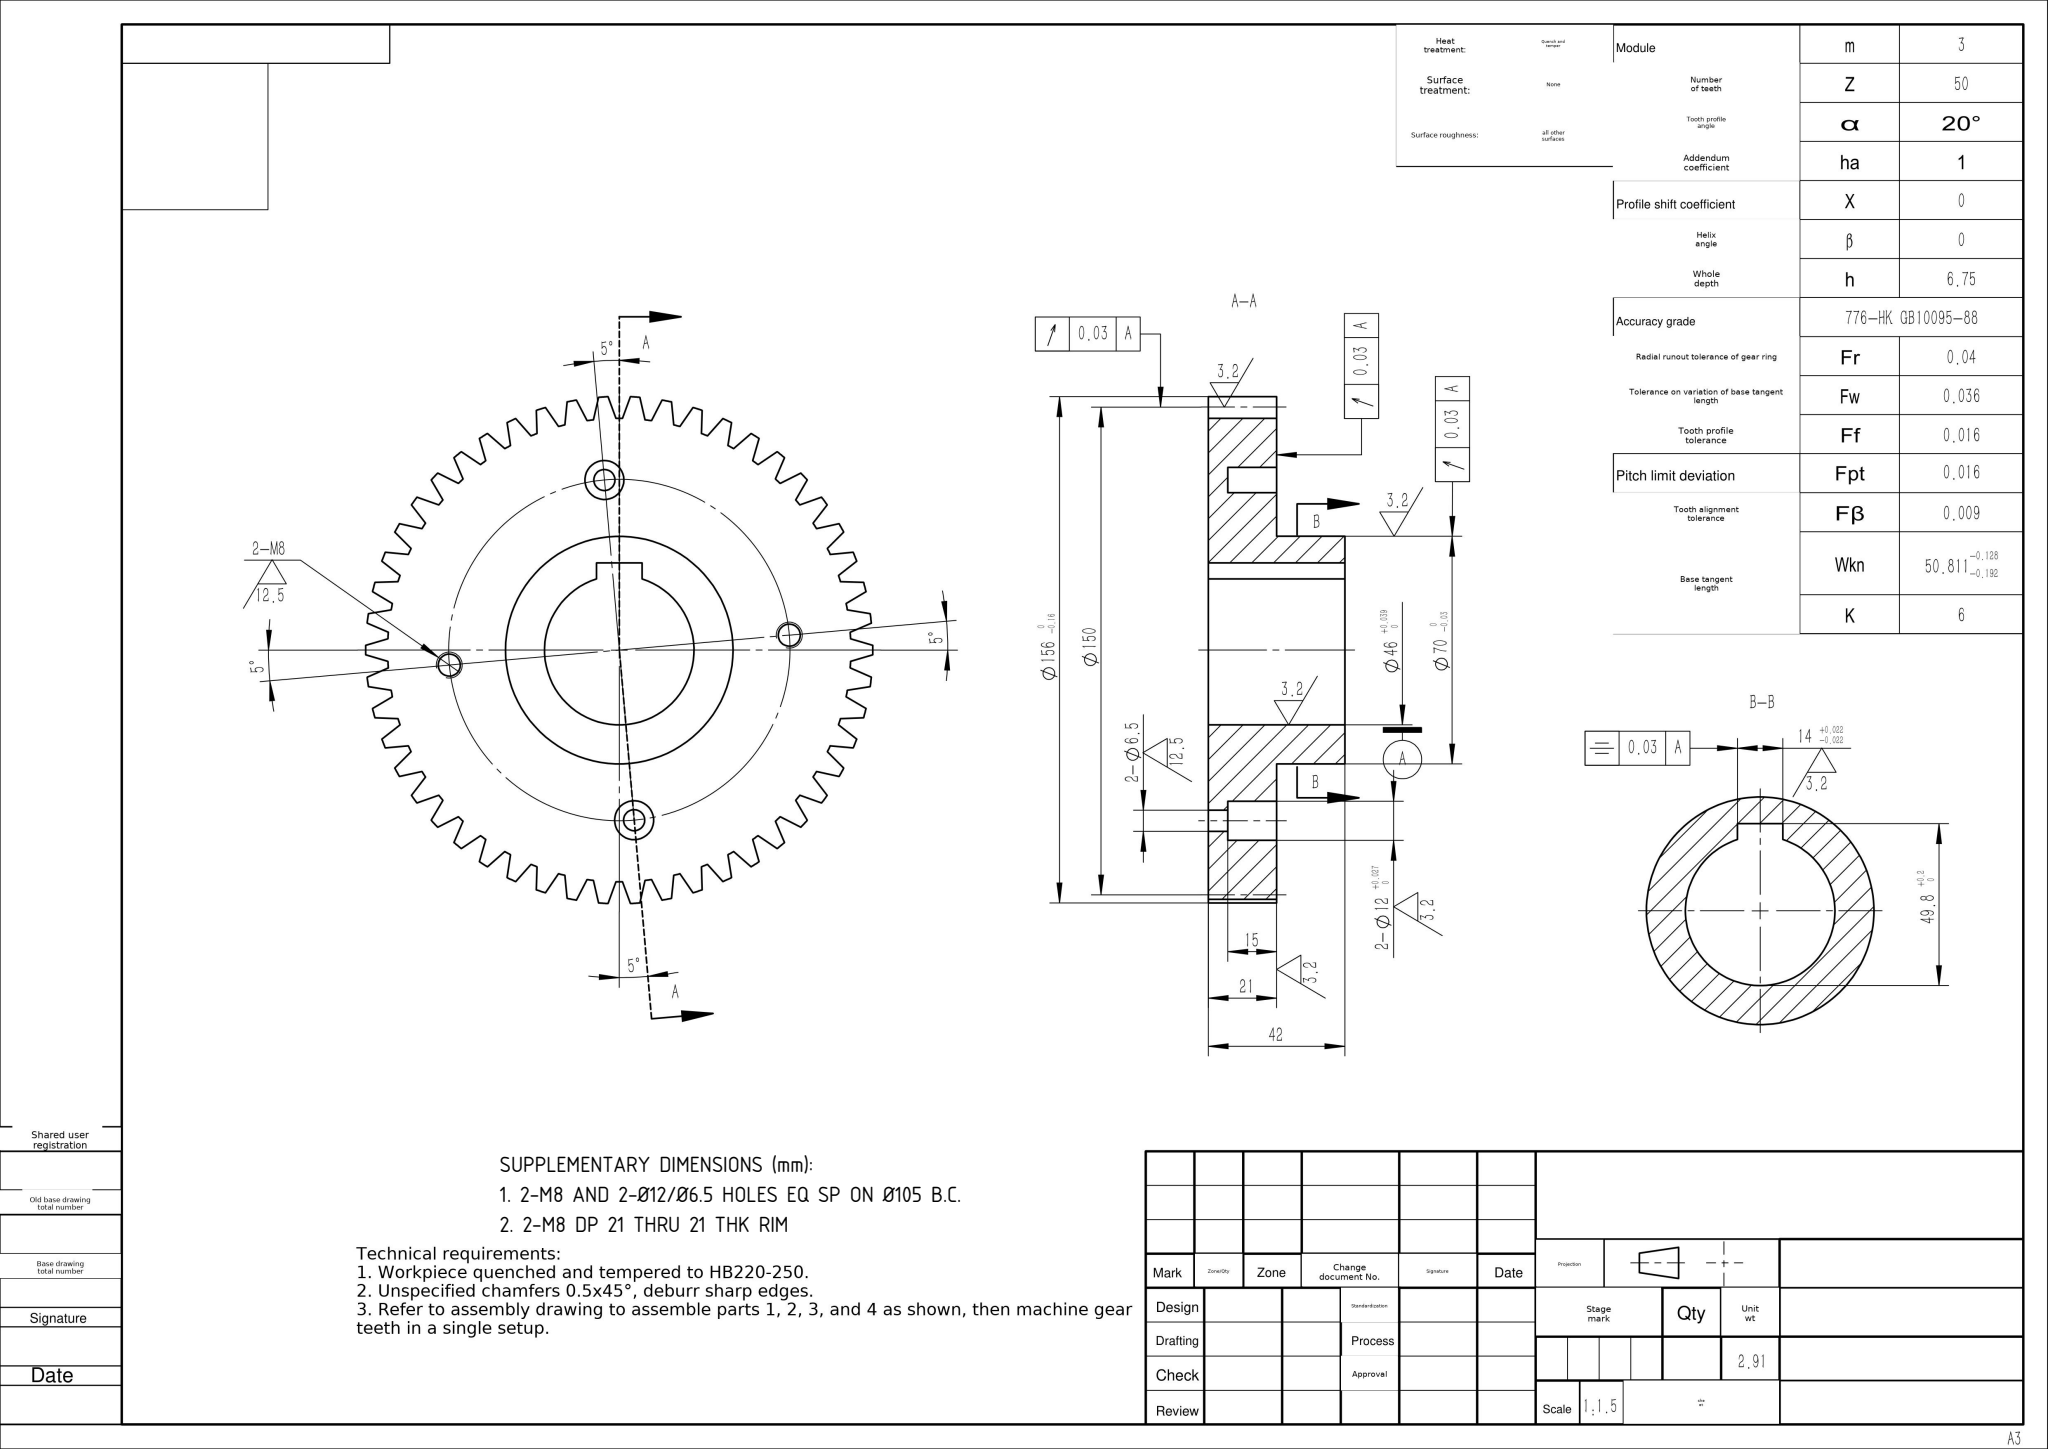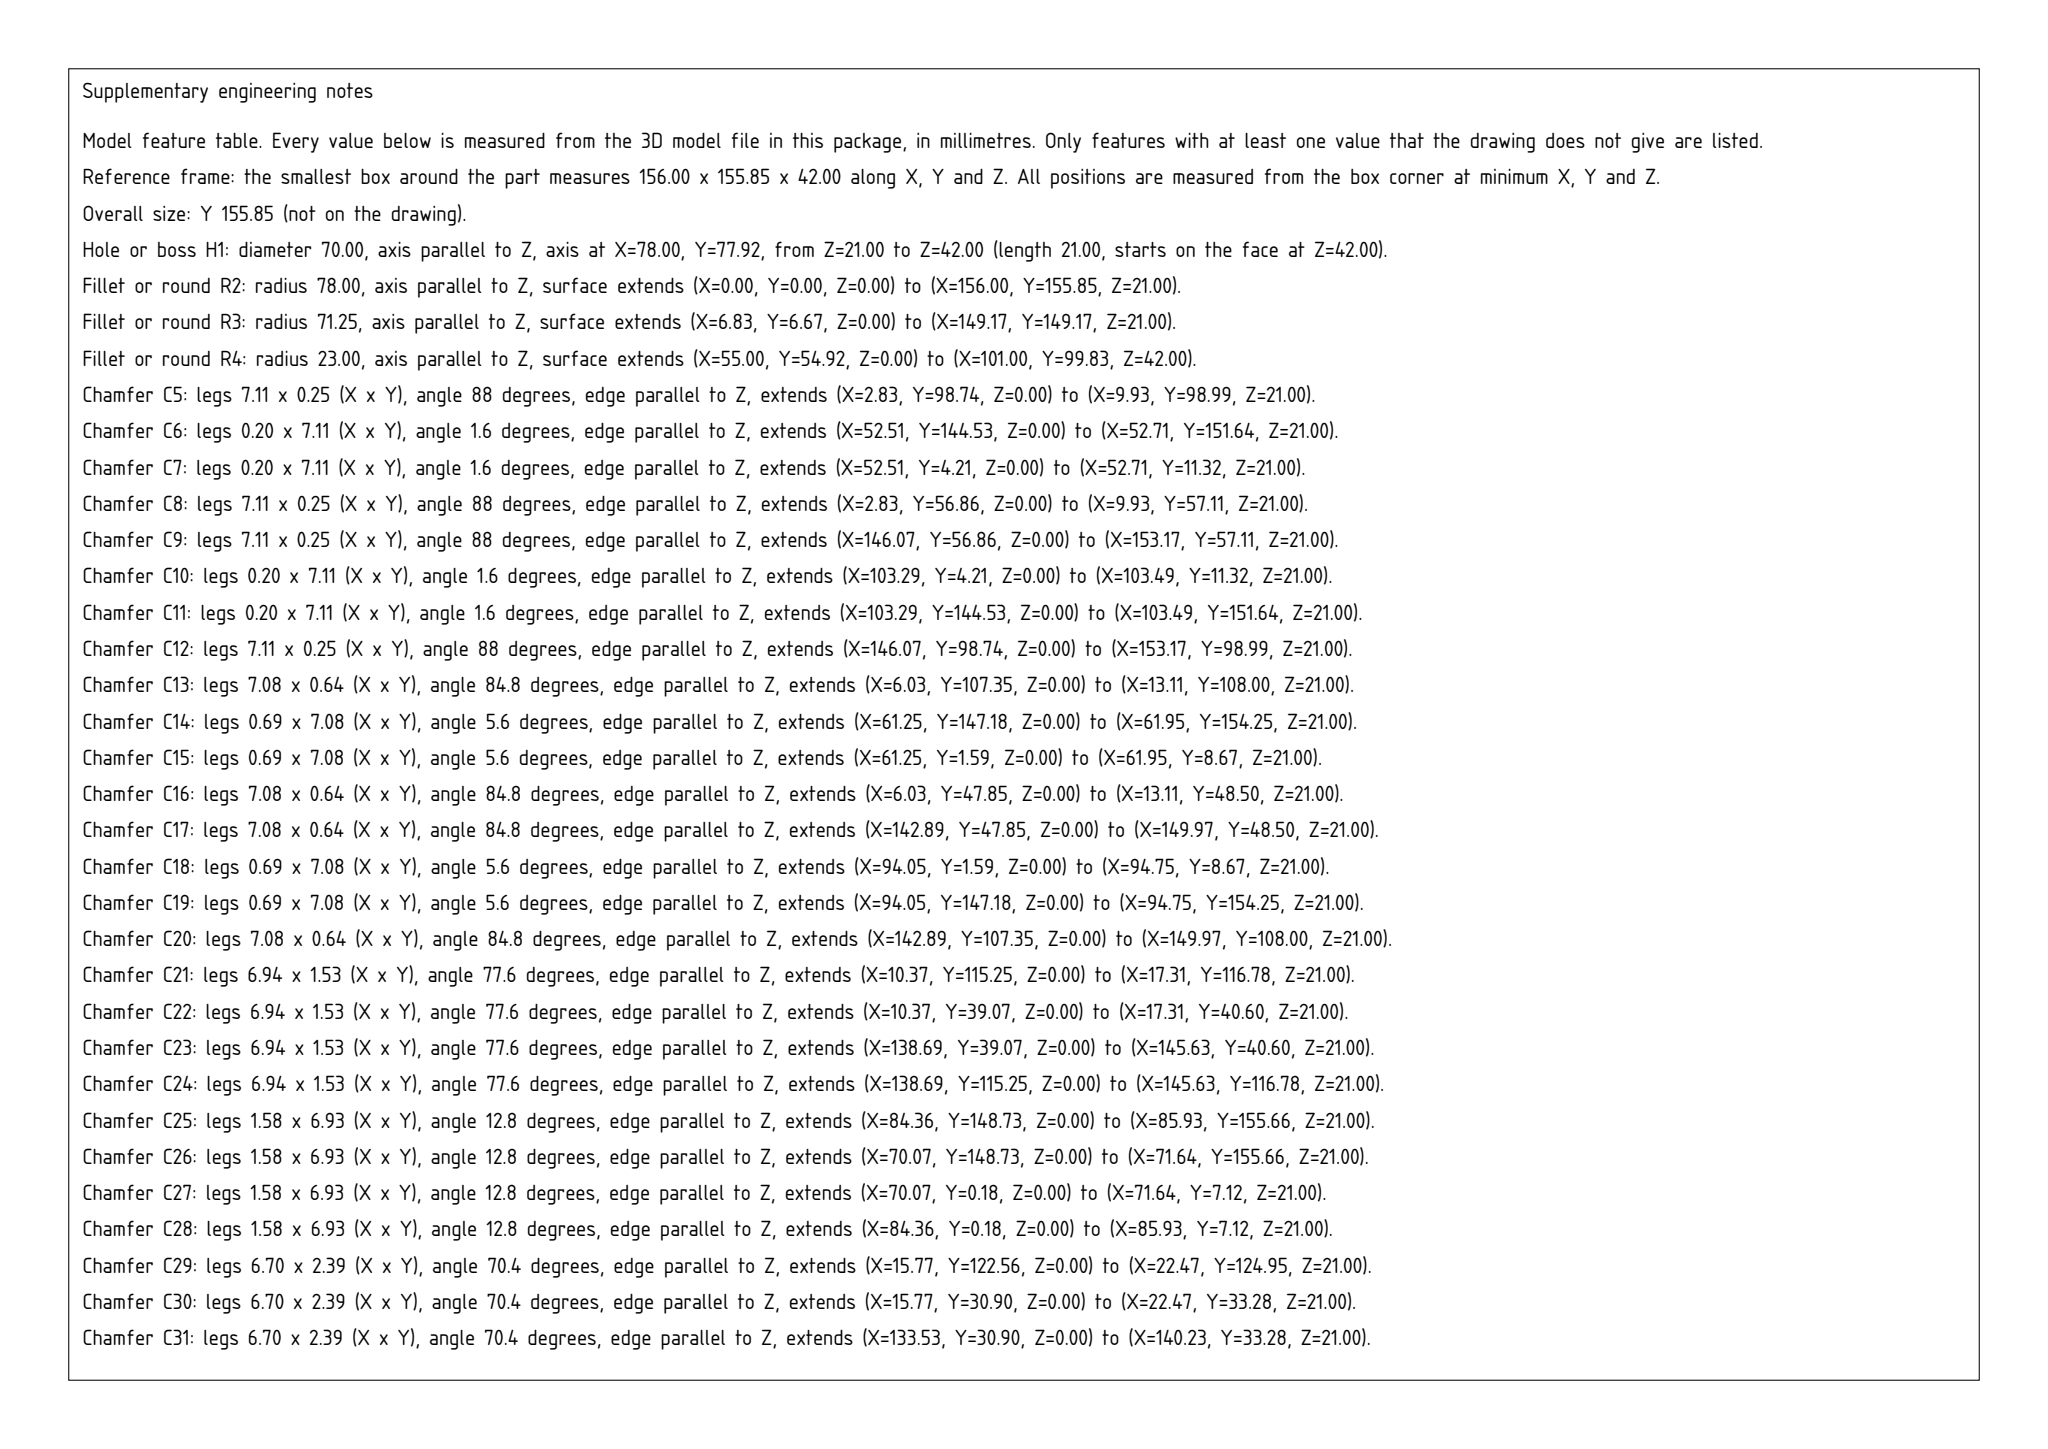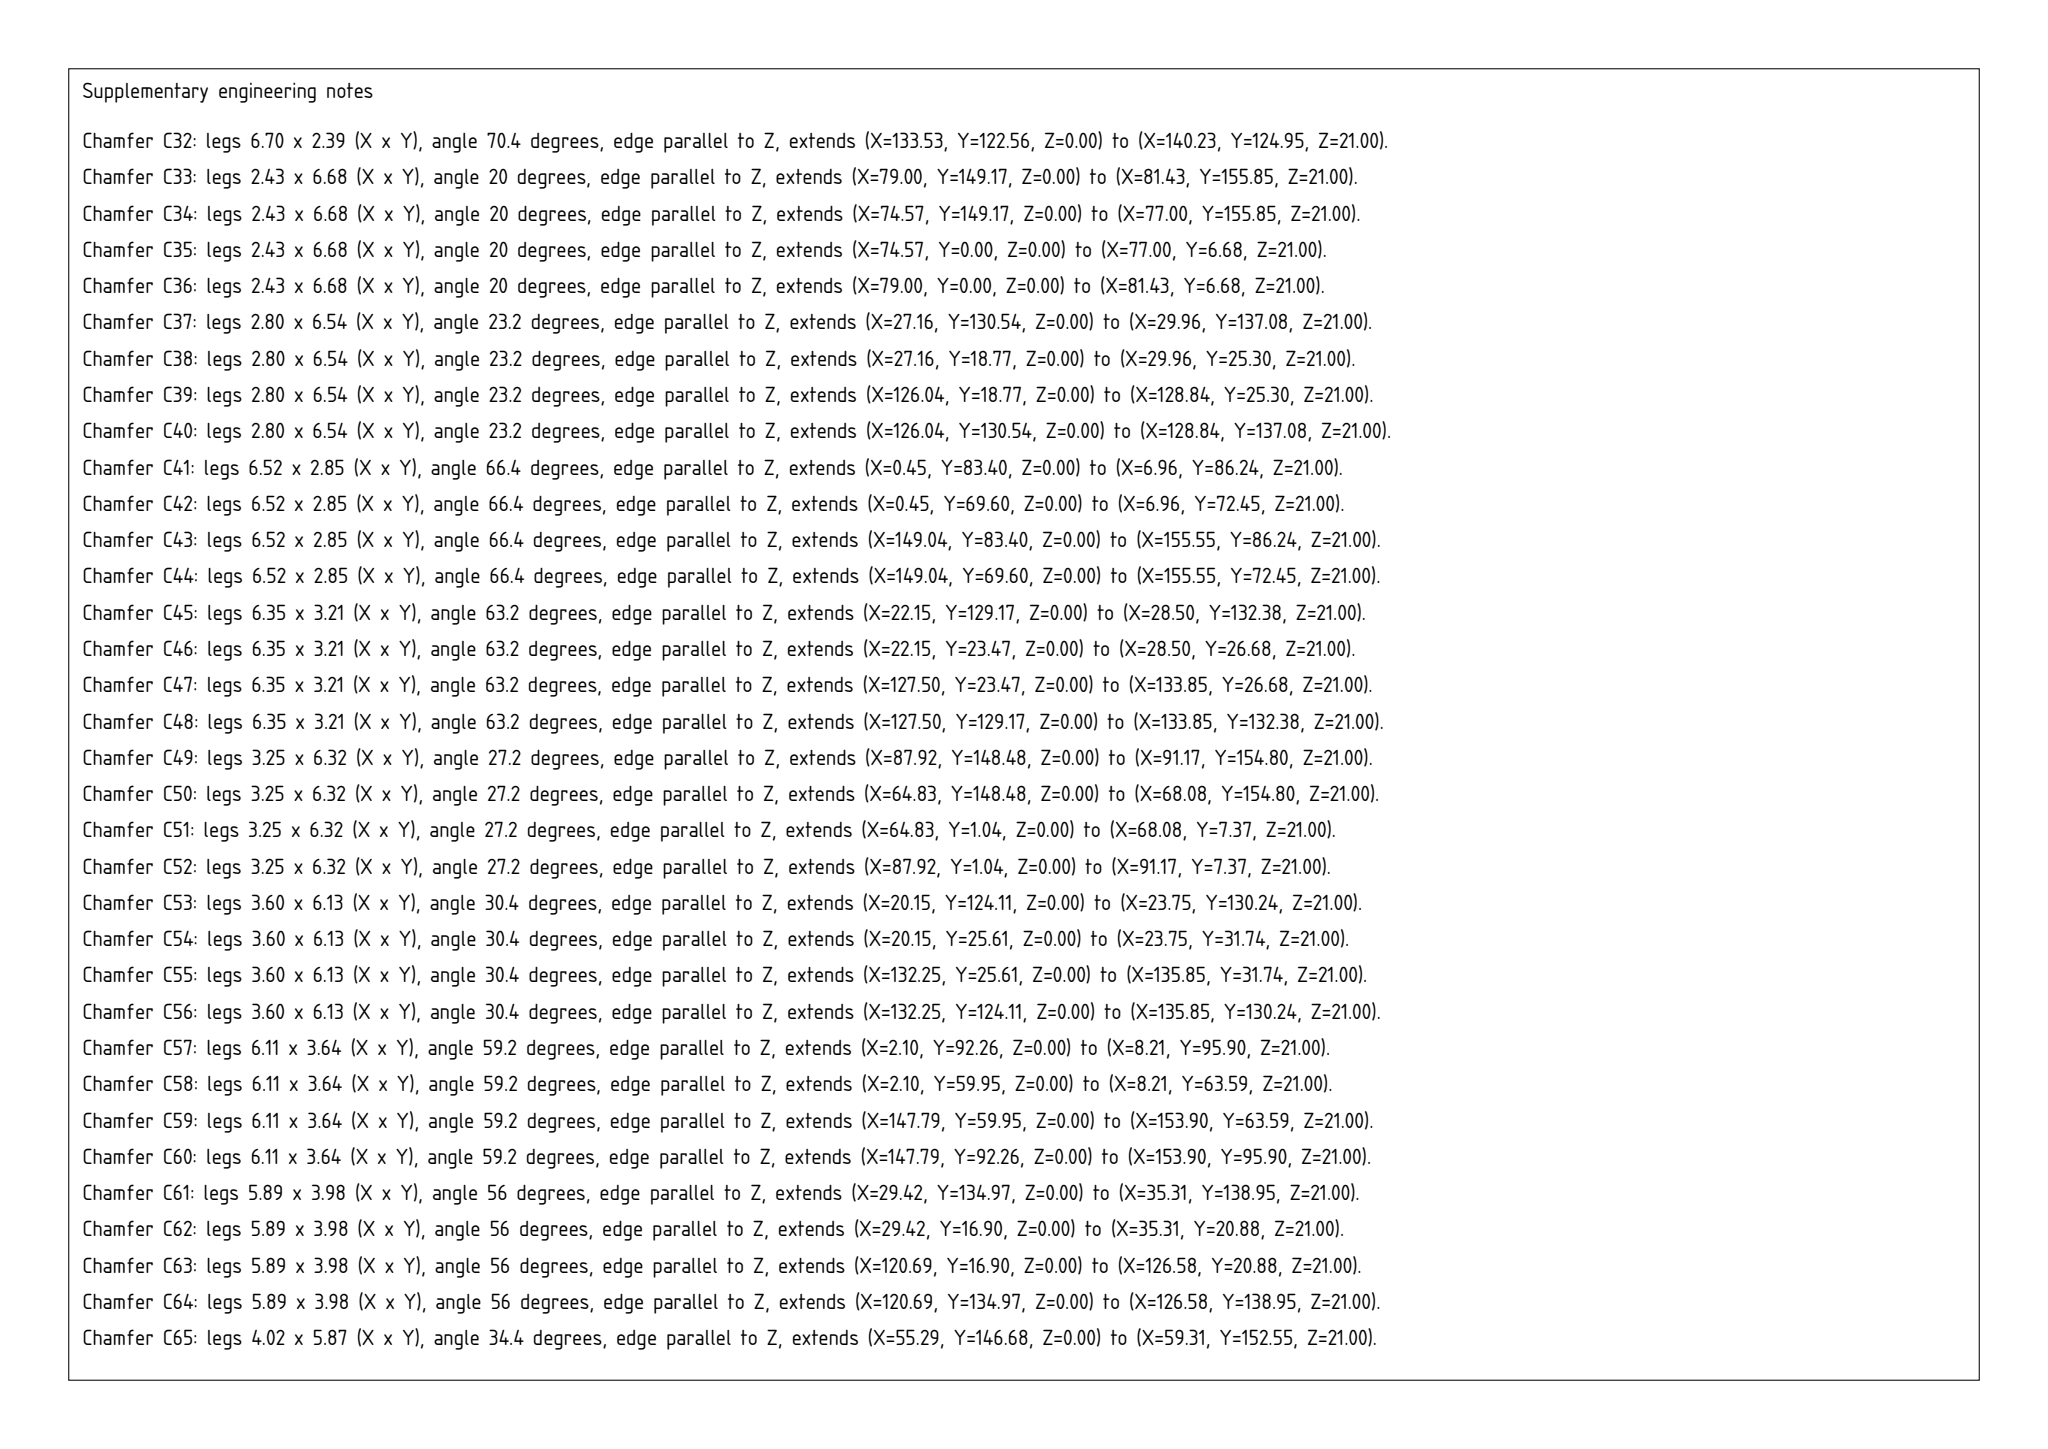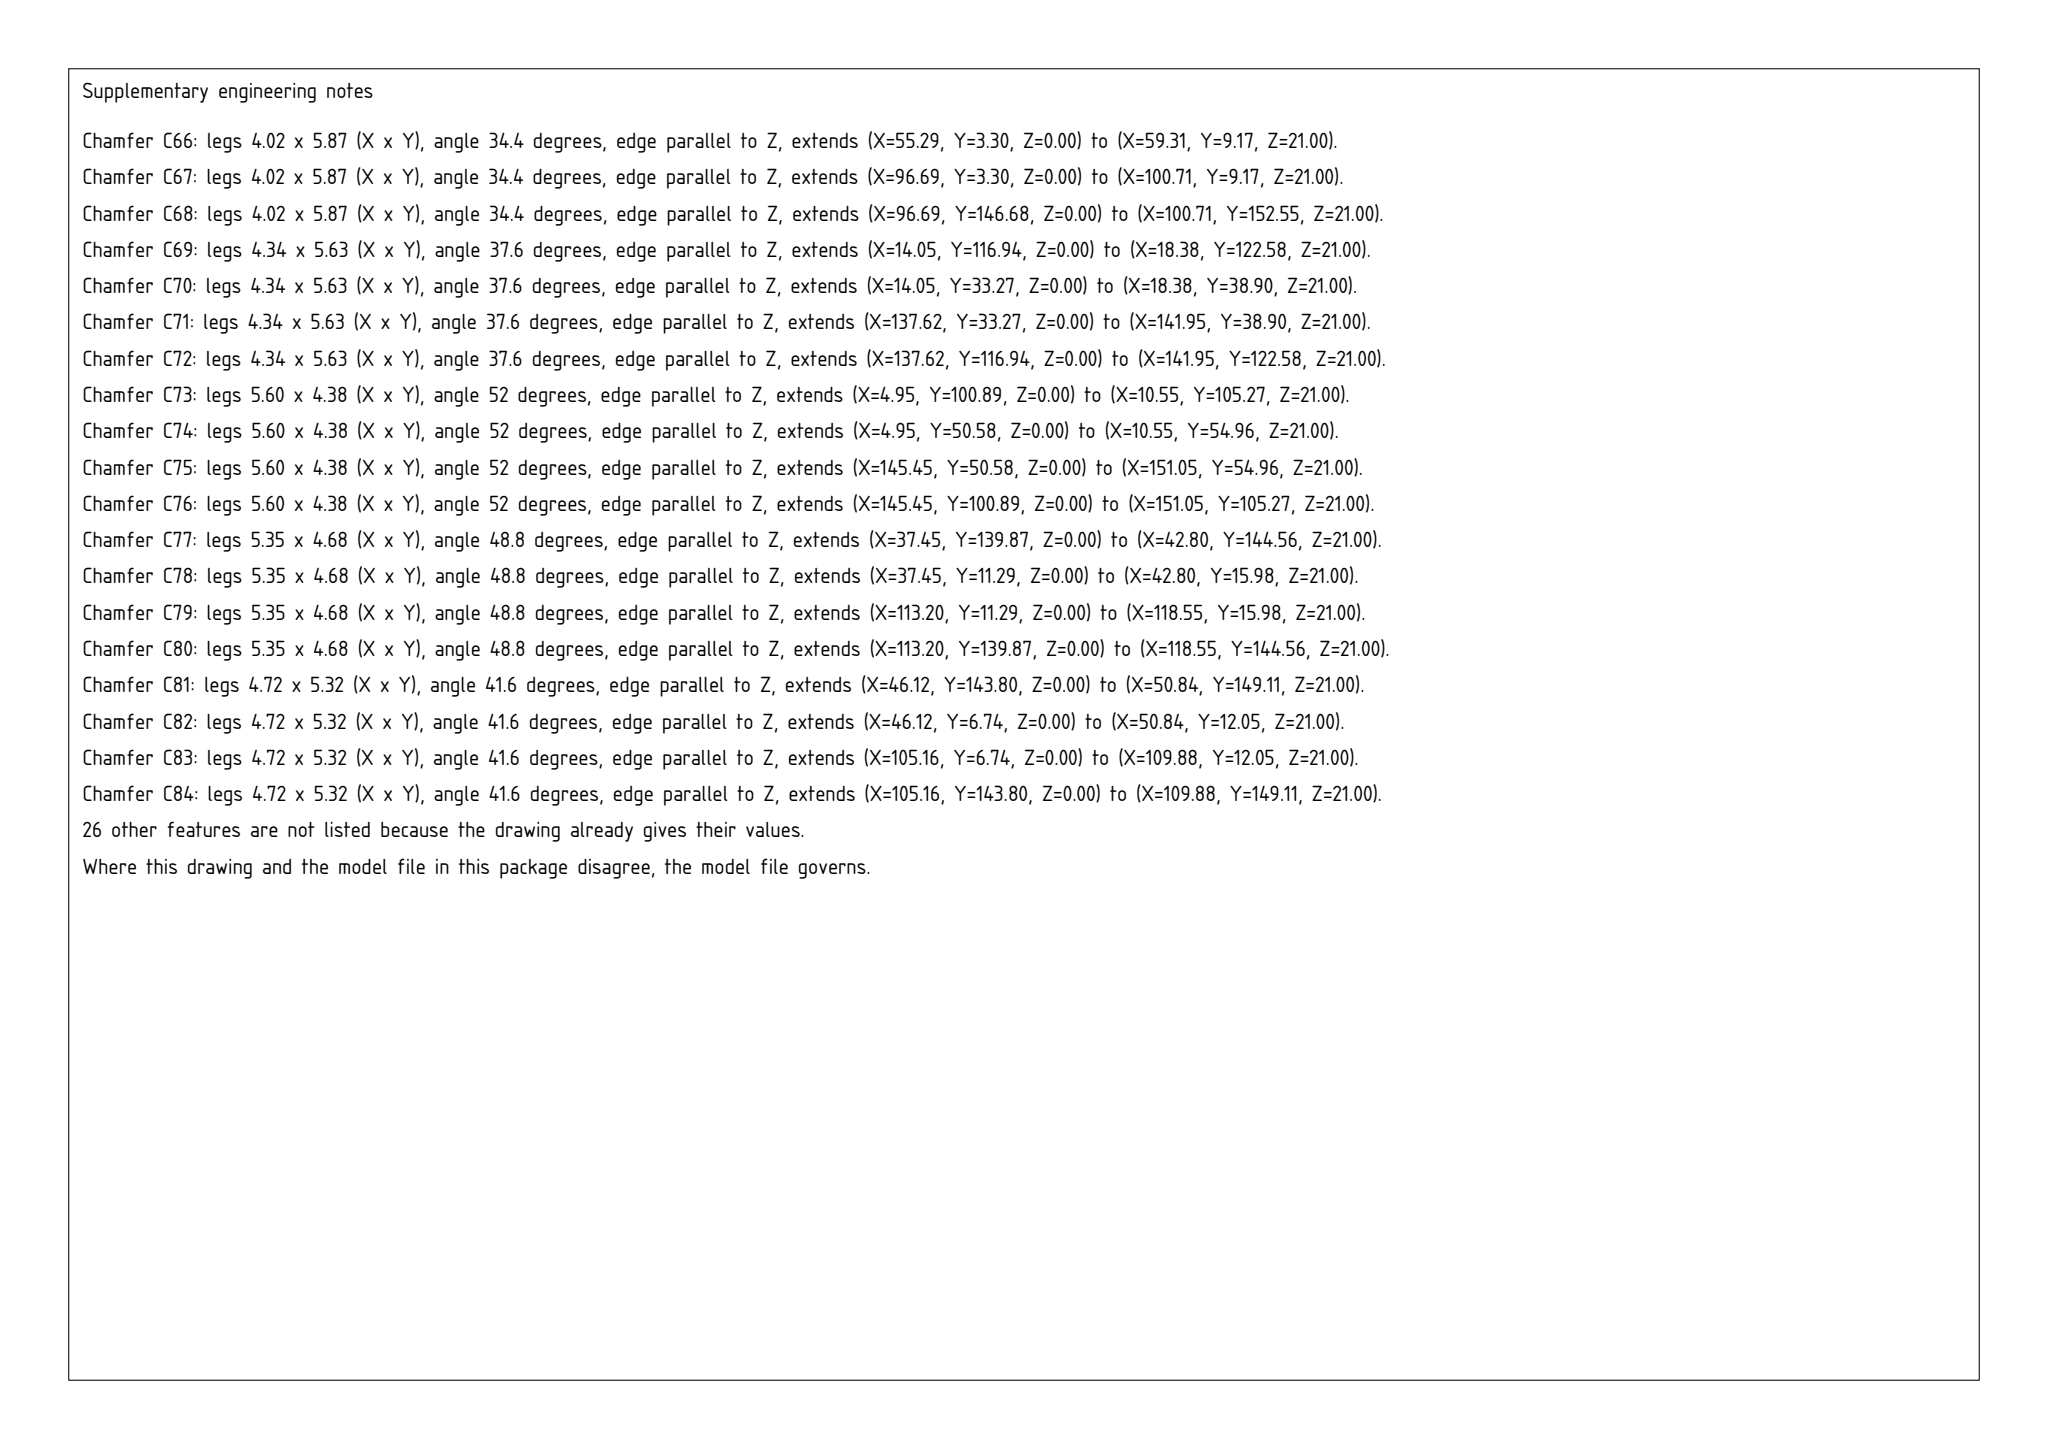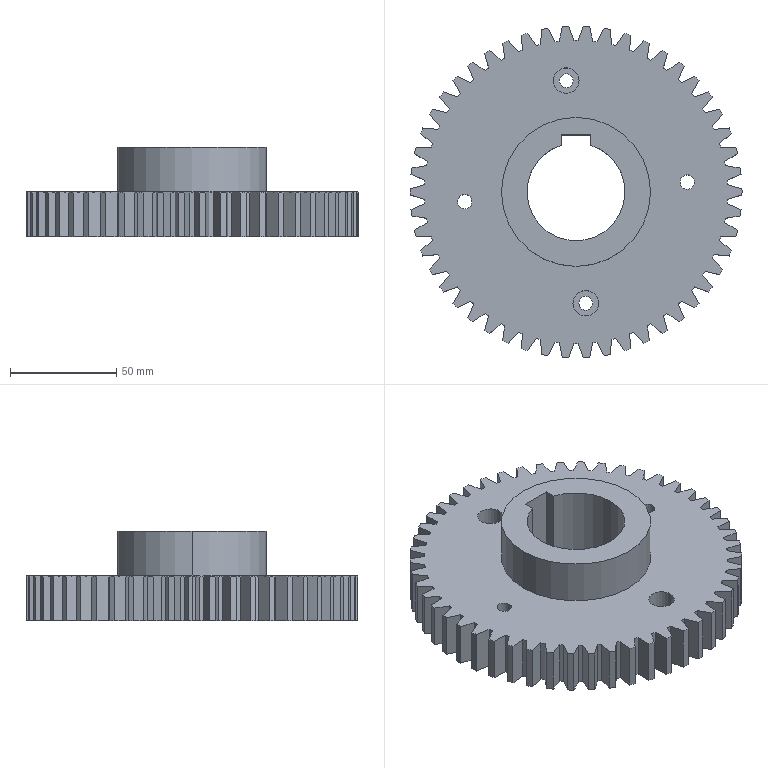Part | SolidWorks | mm | 1 solid | 226 faces | box 156 x 155.85 x 42 mm | volume 373161 mm3 | cylinder 118 | plane 108 | commonest cylinder face diameters 156 x51 142.5 x50 6.5 x4 12 x4 6.8 x4 46 x3 70 x2